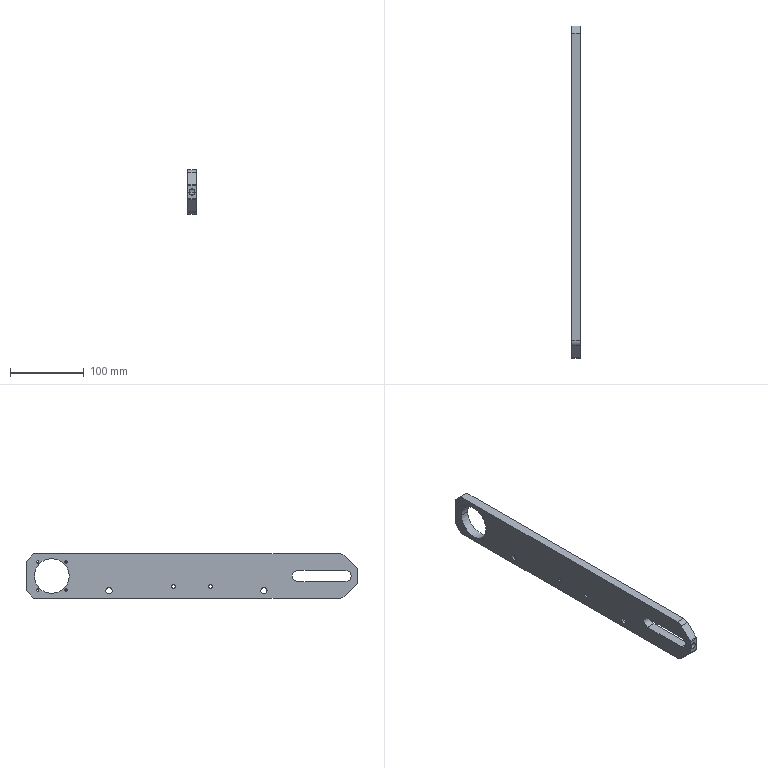Component | SolidWorks | LowerSideBeltXG-XG1-1_LowerRollerMountingPlateBXG-XG1-1 | 1 solid | 45 faces | box 12 x 450 x 60 mm | volume 278920 mm3 | cylinder 31 | plane 14 | commonest cylinder face diameters 3.3 x8 5 x4 14 x4 8.5 x4 15 x3 8.2 x2 47 x2 20 x2
build123d program:
from build123d import *

# Parameters (mm, degrees)
SKETCH1_W               = 450
SKETCH1_H               = 60
SKETCH1_R               = 4.25
SKETCH1_R_2             = 23.5
BOSS_EXTRUDE1_DEPTH     = 6
CHAMFER1_SIZE           = 10
SKETCH5_R               = 7
CUT_EXTRUDE1_DEPTH      = 8.5
CUT_EXTRUDE4_DEPTH      = 228.308
CUT_EXTRUDE5_DEPTH      = 228.308
CUT_EXTRUDE6_REACH      = 453.039
CUT_EXTRUDE6_END_RADIUS = 7.5
SKETCH15_R              = 4.1
FILLET1_R               = 10
FILLET2_R               = 2
CUT_EXTRUDE7_DEPTH      = 228.308
M6_TAPPED_HOLE1_D       = 5
M4_TAPPED_HOLE1_D       = 3.3


with BuildPart() as part:
    # Sketch1 → Boss-Extrude1 (new, symmetric)
    with BuildSketch(Plane.XY):
        Rectangle(SKETCH1_W, SKETCH1_H)
        with Locations((-97.5, -20)):
            Circle(SKETCH1_R, mode=Mode.SUBTRACT)
        with Locations((112.5, -20)):
            Circle(SKETCH1_R, mode=Mode.SUBTRACT)
        with Locations((190, 0)):
            Circle(SKETCH1_R_2, mode=Mode.SUBTRACT)
    extrude(amount=BOSS_EXTRUDE1_DEPTH, both=True)

    # Chamfer1
    chamfer1_edges = [part.edges().sort_by_distance(p)[0] for p in [
        (225, -30, 0),
        (-225, -30, 0),
        (-225, 30, 0),
        (225, 30, 0),
    ]]
    chamfer(chamfer1_edges, length=CHAMFER1_SIZE)

    # Sketch5 → Cut-Extrude1 (cut)
    with BuildSketch(Plane.XY.offset(6)):
        with Locations((-97.5, -20)):
            Circle(SKETCH5_R)
        with Locations((112.5, -20)):
            Circle(SKETCH5_R)
    extrude(amount=-CUT_EXTRUDE1_DEPTH, mode=Mode.SUBTRACT)

    # Sketch12 → Cut-Extrude4 (cut, through all)
    with BuildSketch(Plane.XY.offset(6)):
        with BuildLine():
            Line((-208.5, 7.5), (-148.5, 7.5))
            ThreePointArc((-148.5, 7.5), (-141, 0), (-148.5, -7.5))
            Line((-148.5, -7.5), (-208.5, -7.5))
            ThreePointArc((-208.5, -7.5), (-216, 0), (-208.5, 7.5))
        make_face()
    extrude(amount=-CUT_EXTRUDE4_DEPTH, mode=Mode.SUBTRACT)

    # Sketch14 → Cut-Extrude5 (cut, symmetric)
    with BuildSketch(Plane.XY.offset(6)):
        Polygon((440.976, 675.976), (-205, 30), (-225, 10), (-870.976, -635.976), (-2162.929, 655.976), (-850.976, 1967.929), align=None)
    cut_extrude5 = extrude(amount=CUT_EXTRUDE5_DEPTH, both=True, mode=Mode.SUBTRACT)

    # Mirror1: Cut-Extrude5 across plane
    add(cut_extrude5.mirror(Plane.ZX), mode=Mode.SUBTRACT)

    # Cut-Extrude6: up to this cylinder (the profile starts outside it)
    cut_extrude6_end = Plane(origin=(-208.5, 0, 0), z_dir=(0, 0, 1)) * Cylinder(CUT_EXTRUDE6_END_RADIUS, 922.078, mode=Mode.PRIVATE)
    # Sketch15 → Cut-Extrude6 (cut, up to the surface)
    with BuildSketch(Plane.ZY.offset(225), mode=Mode.PRIVATE) as cut_extrude6_sk1:
        Circle(SKETCH15_R)
    cut_extrude6_tool1 = extrude(cut_extrude6_sk1.sketch, amount=-CUT_EXTRUDE6_REACH, mode=Mode.PRIVATE) - cut_extrude6_end
    add(cut_extrude6_tool1.solids().sort_by_distance((-225, 0, 0))[0], mode=Mode.SUBTRACT)

    # Fillet1
    fillet1_edges = [part.edges().sort_by_distance(p)[0] for p in [
        (-205, 30, 0),
        (-205, -30, 0),
    ]]
    fillet(fillet1_edges, radius=FILLET1_R)

    # Fillet2
    fillet2_edges = [part.edges().sort_by_distance(p)[0] for p in [
        (-225, 10, 0),
        (-225, -10, 0),
    ]]
    fillet(fillet2_edges, radius=FILLET2_R)

    # Sketch16 → Cut-Extrude7 (cut, through all)
    with BuildSketch(Plane.XY.offset(6)):
        with BuildLine():
            Line((-148.5, 7.5), (-143.5, 7.5))
            ThreePointArc((-143.5, 7.5), (-136, 0), (-143.5, -7.5))
            Line((-143.5, -7.5), (-148.5, -7.5))
            Line((-148.5, -7.5), (-148.5, 7.5))
        make_face()
    extrude(amount=-CUT_EXTRUDE7_DEPTH, mode=Mode.SUBTRACT)

    # M6 Tapped Hole1 (through all)
    with Locations(Plane.XY.offset(6)):
        with Locations((-25, -14), (25, -14)):
            Hole(M6_TAPPED_HOLE1_D / 2)

    # M4 Tapped Hole1 (through all)
    with Locations(Plane.XY.offset(6)):
        with Locations((170.908, 19.092), (209.092, 19.092), (209.092, -19.092), (170.908, -19.092)):
            Hole(M4_TAPPED_HOLE1_D / 2)


solid = part.part

# Placed as in the assembly
solid = solid.moved(Location((-190.22, 435, 114), (90, 90, 0)))